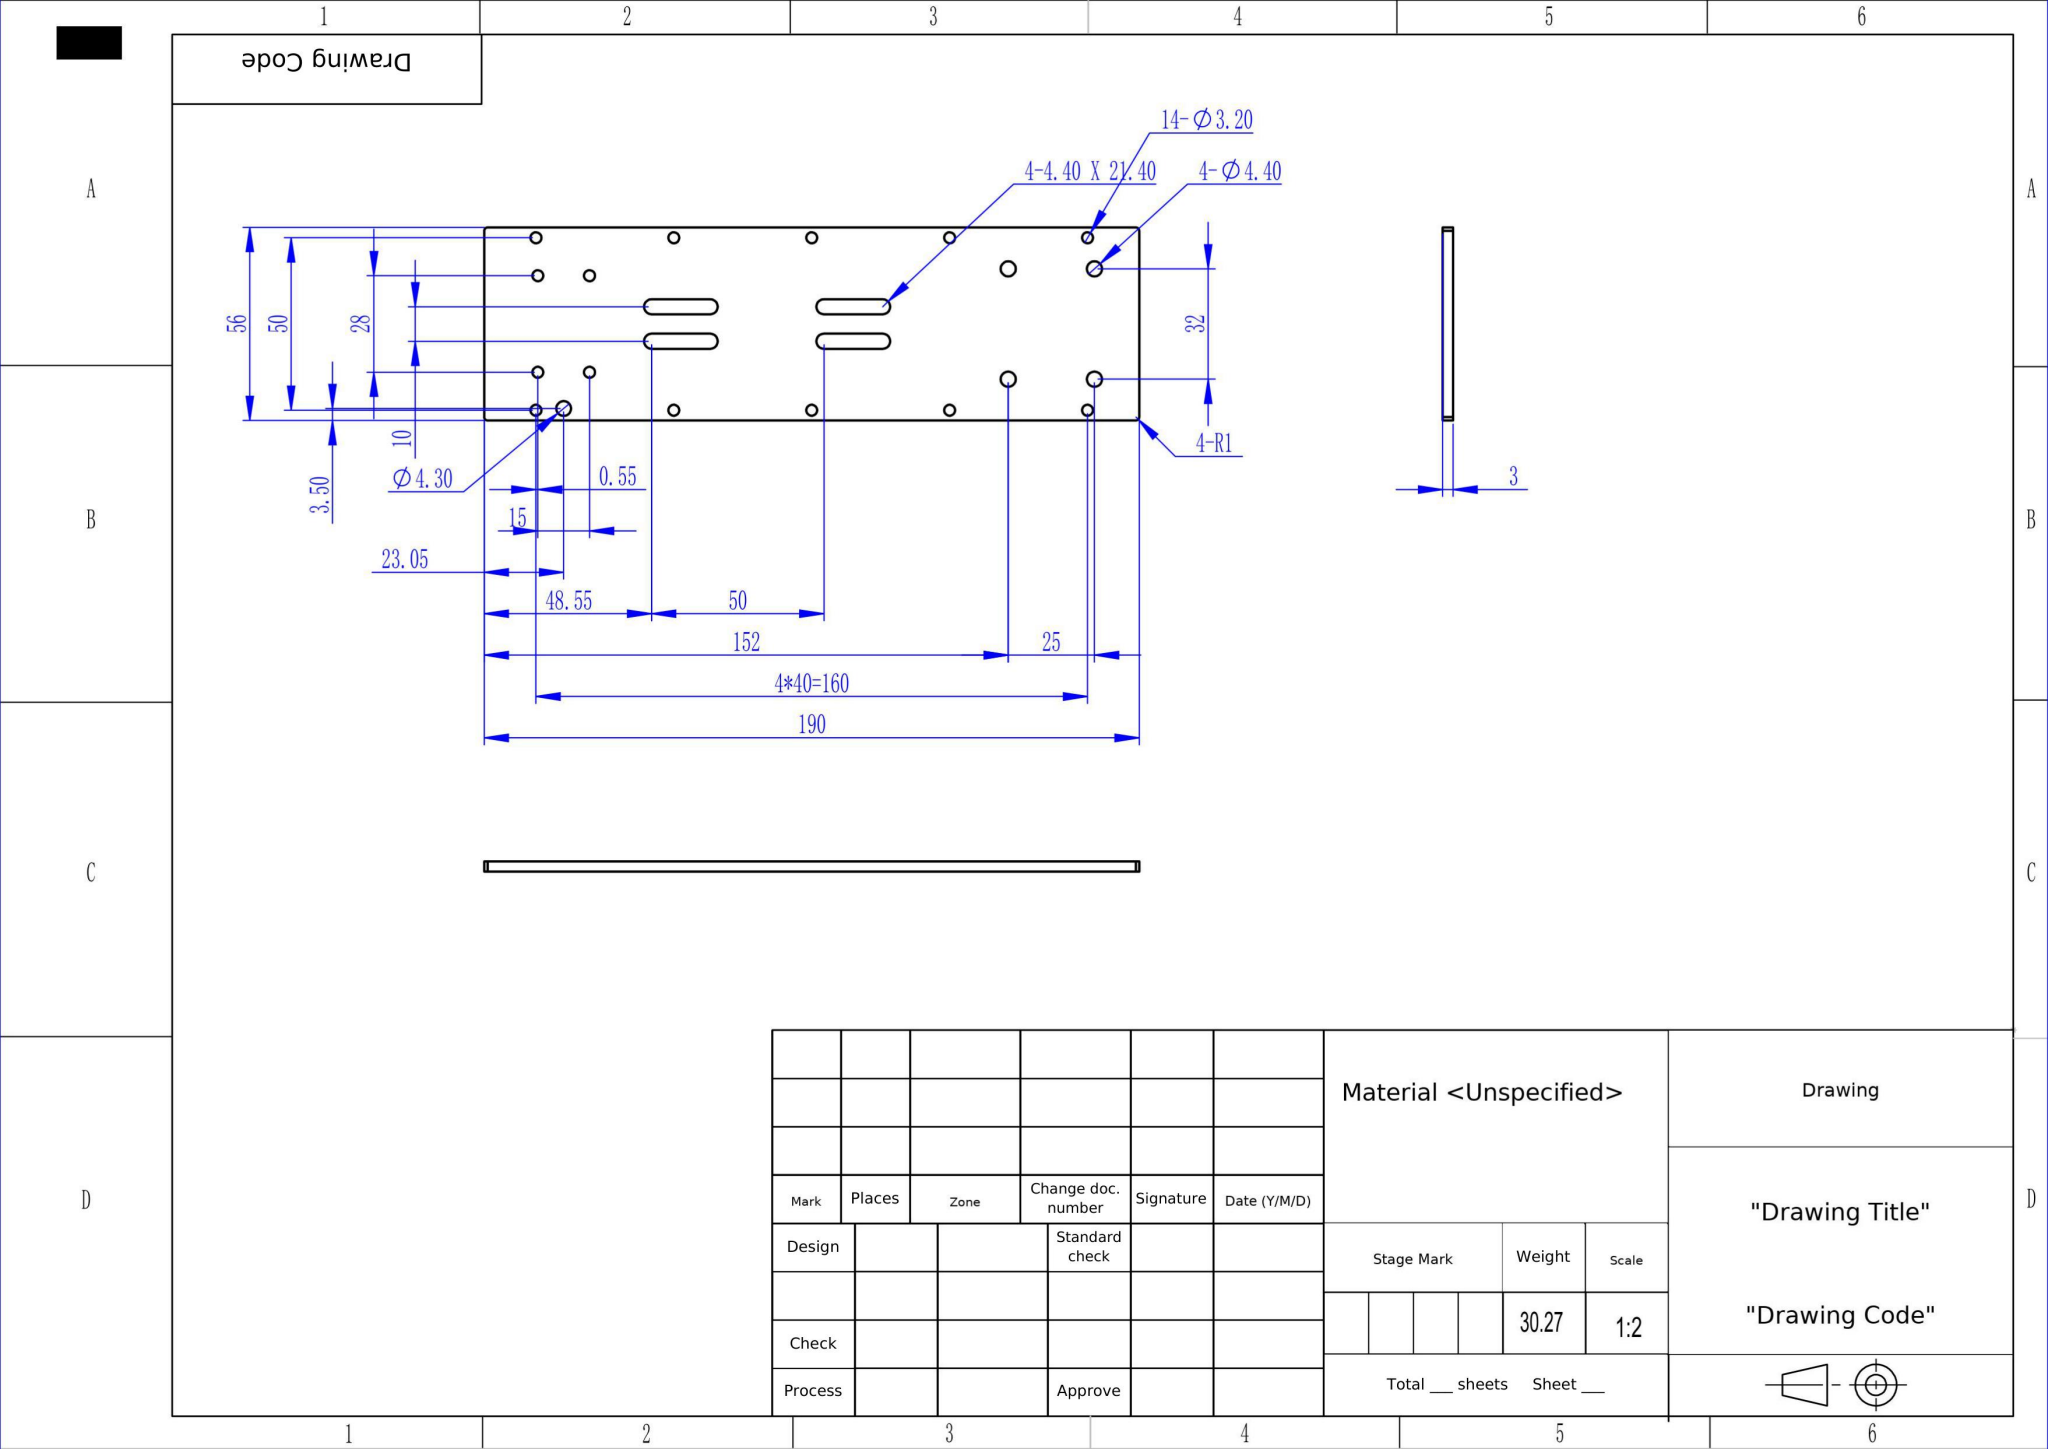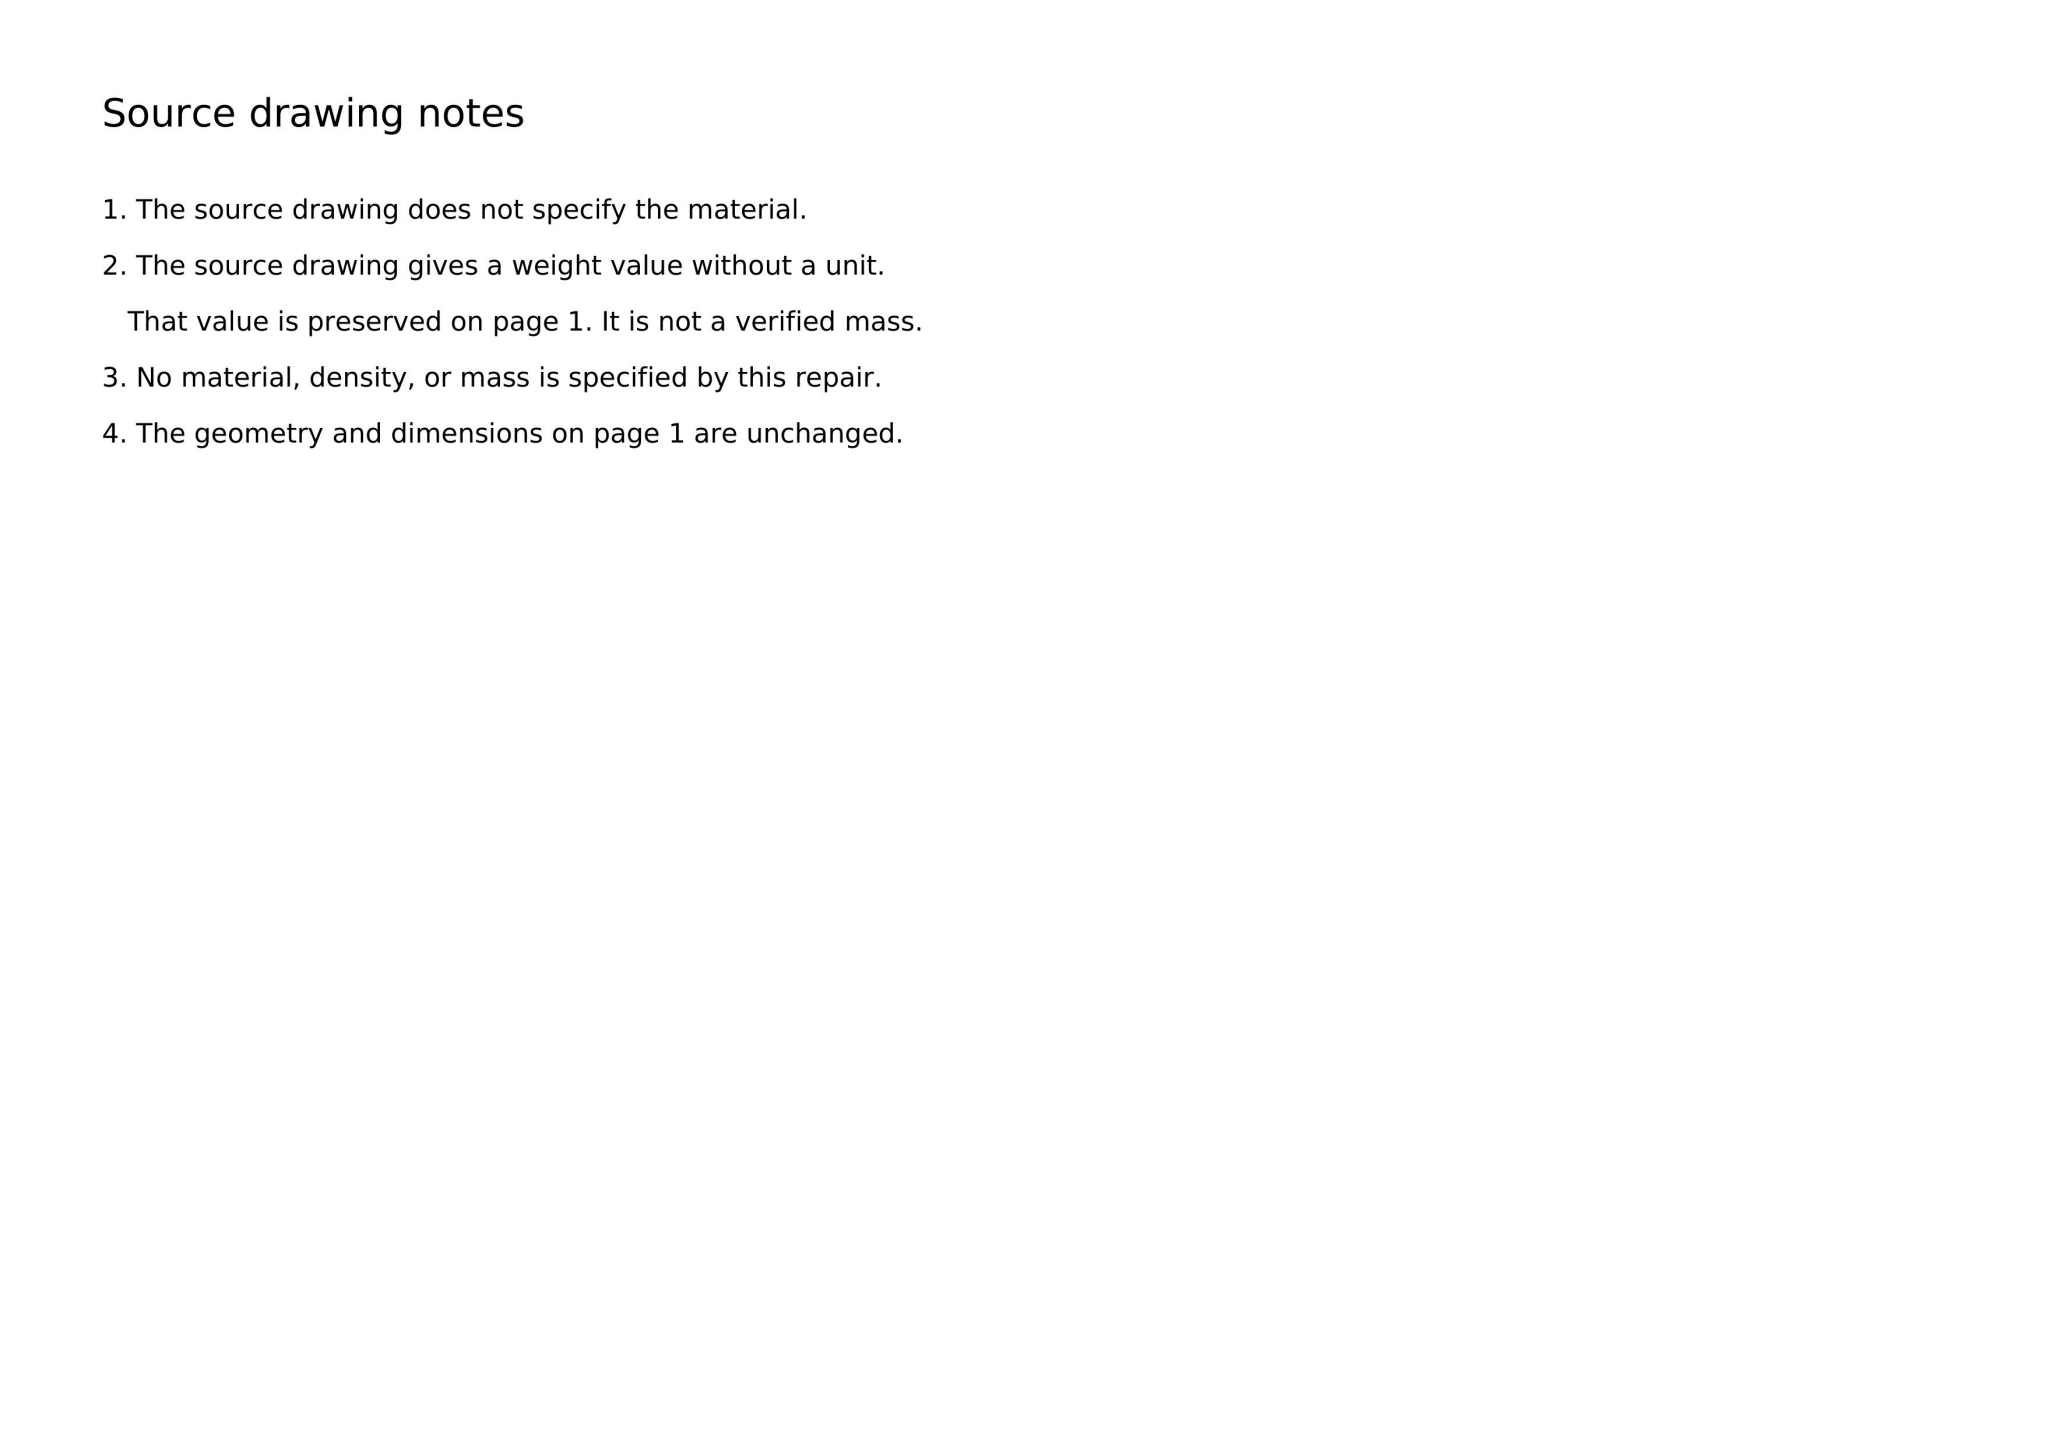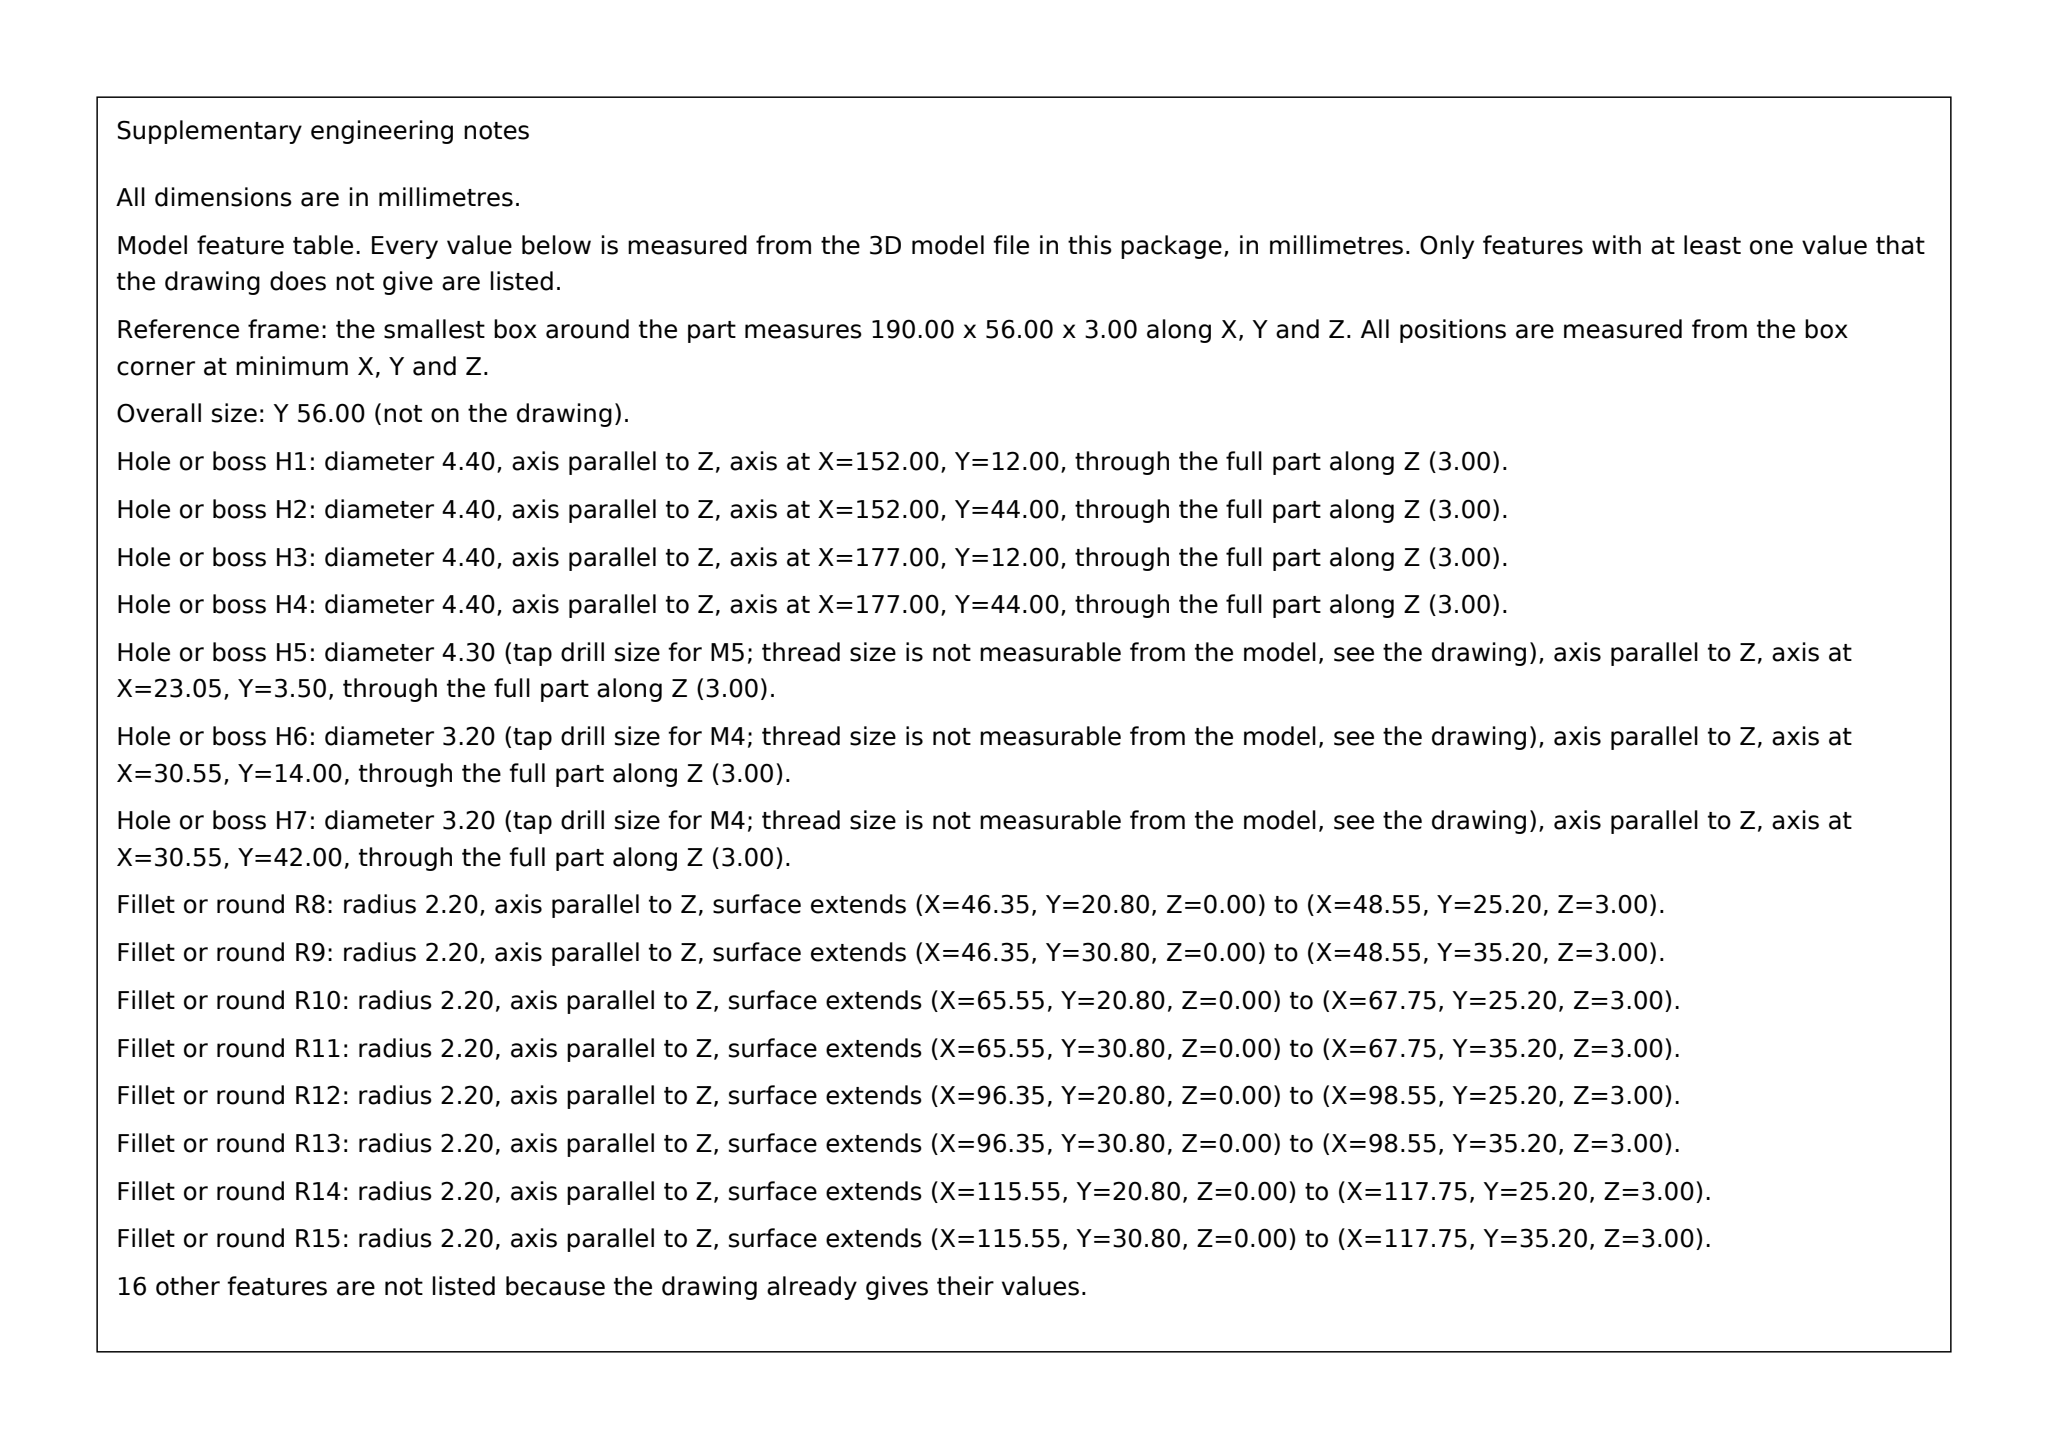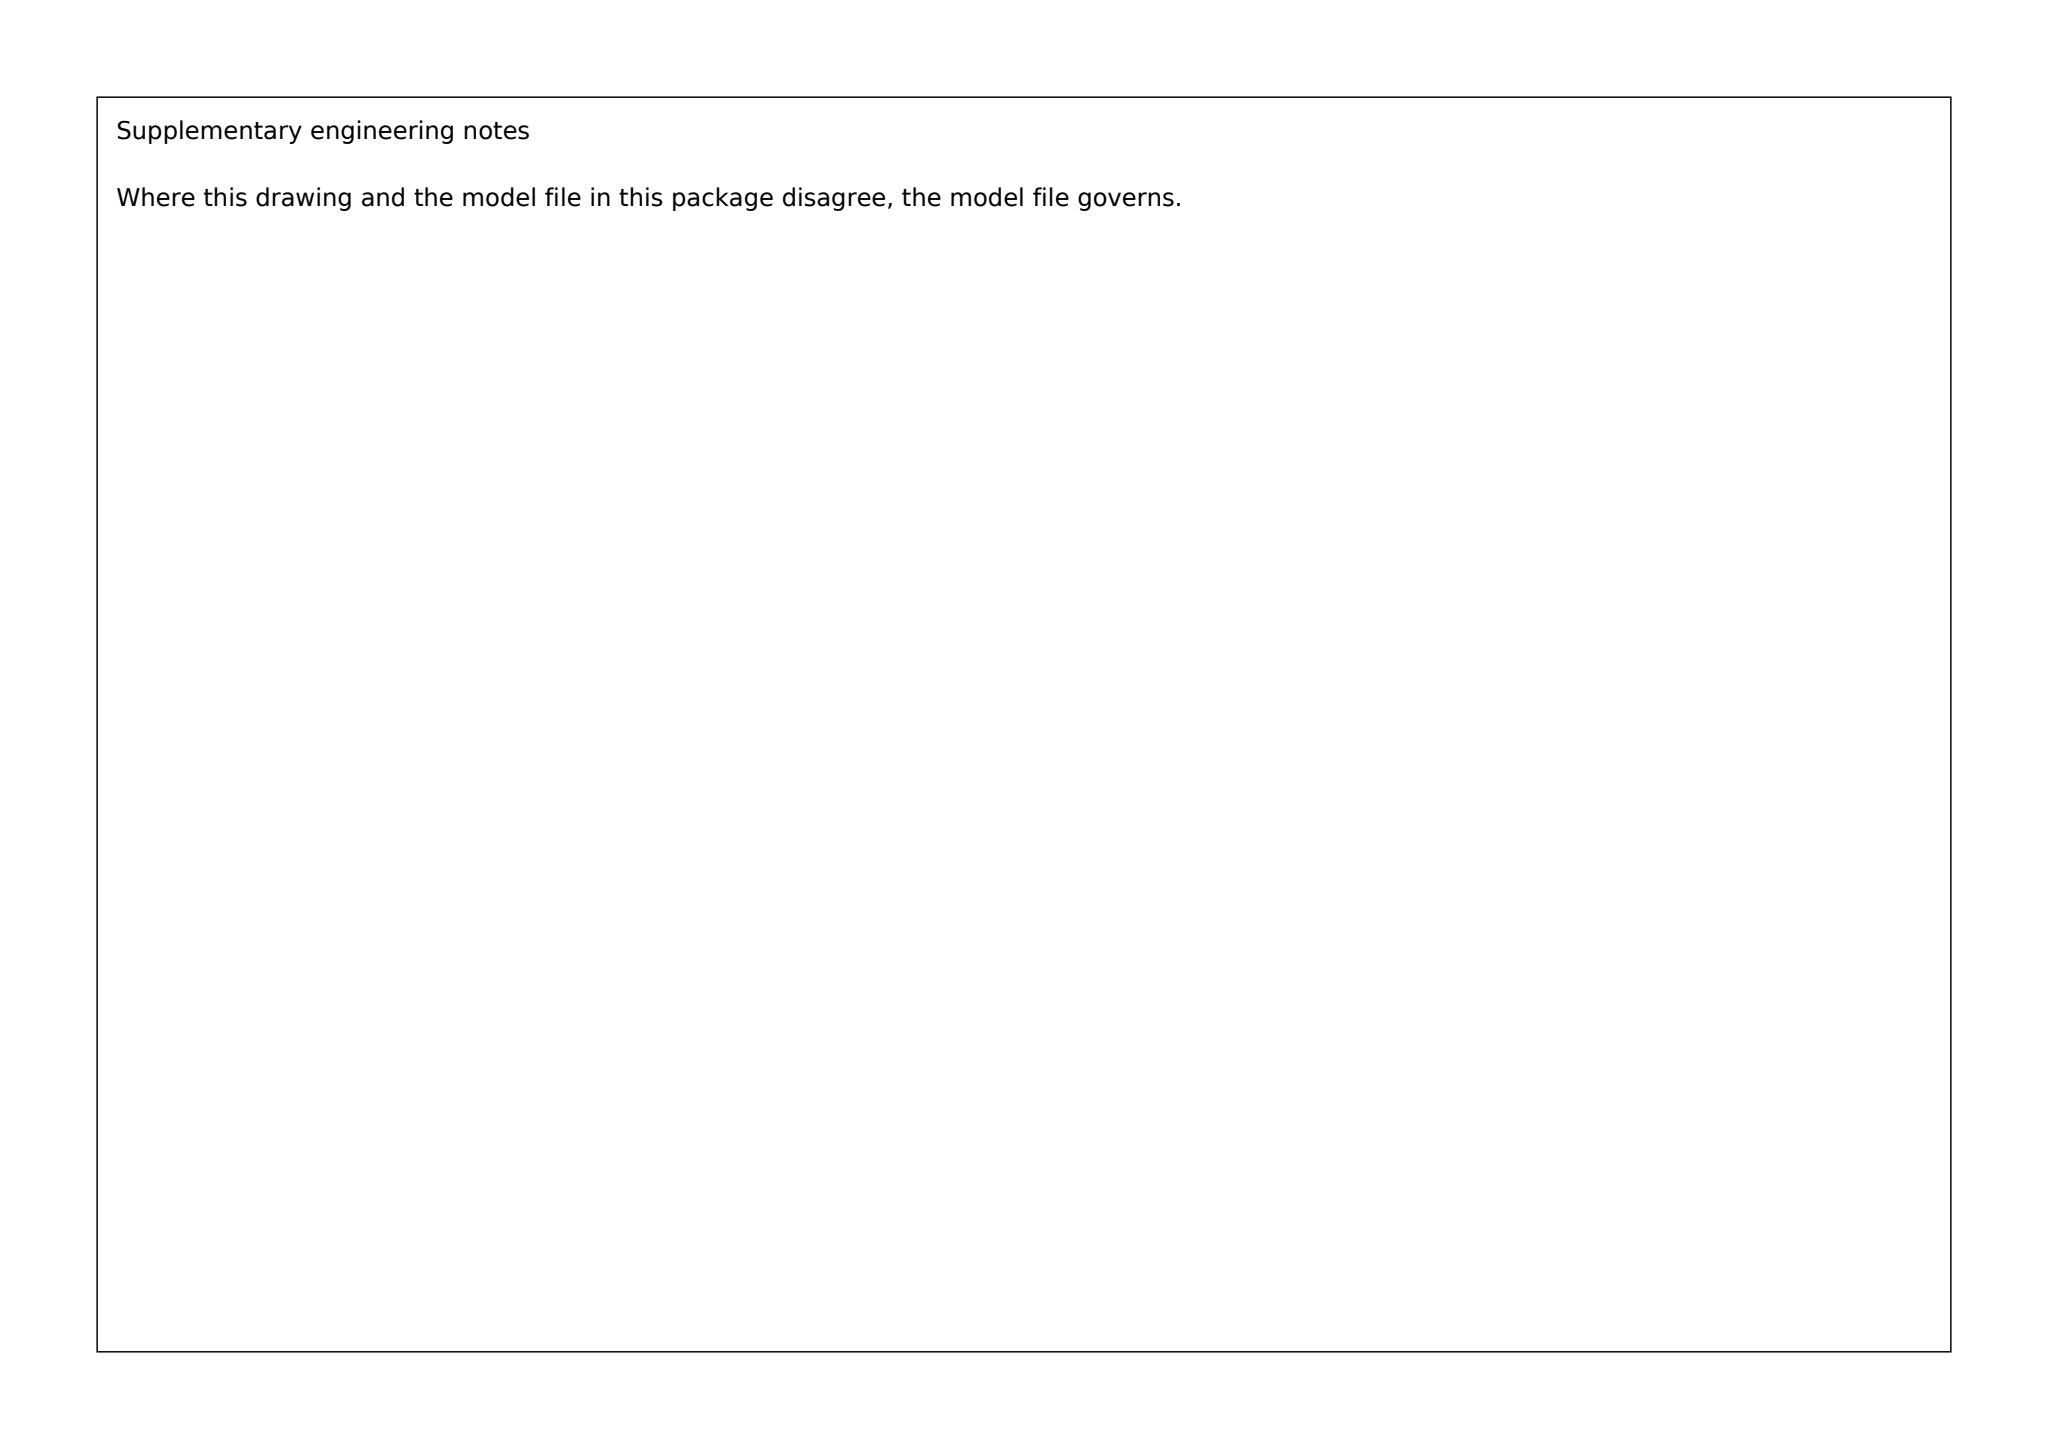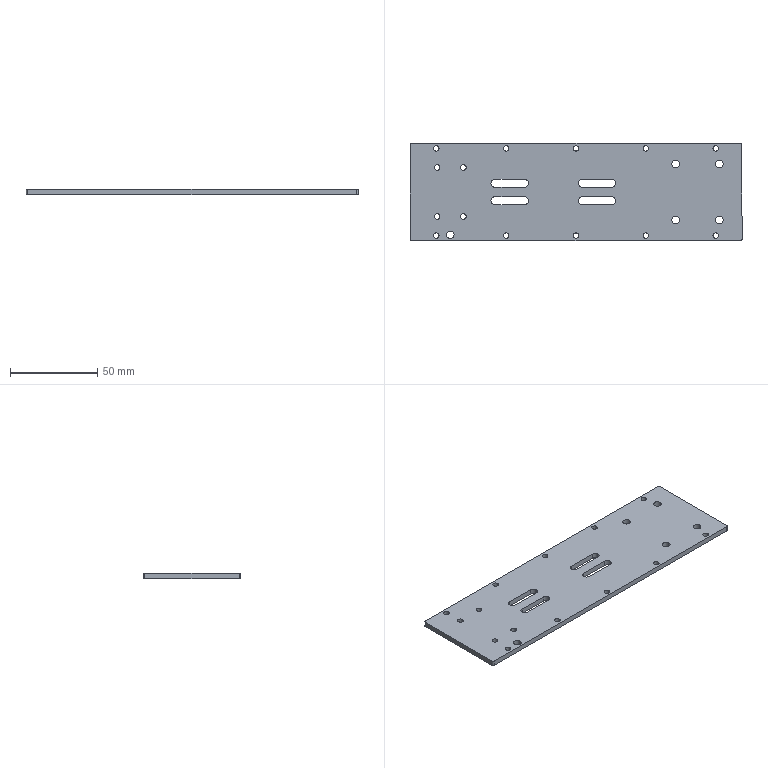Part | SolidWorks | mm | 1 solid | 72 faces | box 190 x 56 x 3 mm | volume 30274 mm3 | cylinder 58 | plane 14 | commonest cylinder face diameters 3.2 x28 4.4 x24 2 x4 4.3 x2
build123d program:
from build123d import *

# Parameters (mm, degrees)
SKETCH1_W           = 190
SKETCH1_H           = 56
SKETCH1_R           = 1.6
SKETCH1_R_2         = 2.2
SKETCH1_R_3         = 2.15
BOSS_EXTRUDE1_DEPTH = 3
FILLET1_R           = 1
CUT_EXTRUDE1_DEPTH  = 193.076


with BuildPart() as part:
    # Sketch1 → Boss-Extrude1 (new body)
    with BuildSketch(Plane.XY):
        with Locations((95, 0)):
            Rectangle(SKETCH1_W, SKETCH1_H)
        with Locations((30.55, 14)):
            Circle(SKETCH1_R, mode=Mode.SUBTRACT)
        with Locations((15.55, 14)):
            Circle(SKETCH1_R, mode=Mode.SUBTRACT)
        with Locations((15.55, -14)):
            Circle(SKETCH1_R, mode=Mode.SUBTRACT)
        with Locations((30.55, -14)):
            Circle(SKETCH1_R, mode=Mode.SUBTRACT)
        with Locations((177, 16)):
            Circle(SKETCH1_R_2, mode=Mode.SUBTRACT)
        with Locations((152, 16)):
            Circle(SKETCH1_R_2, mode=Mode.SUBTRACT)
        with Locations((152, -16)):
            Circle(SKETCH1_R_2, mode=Mode.SUBTRACT)
        with Locations((177, -16)):
            Circle(SKETCH1_R_2, mode=Mode.SUBTRACT)
        with Locations((48.55, 5)):
            Circle(SKETCH1_R_2, mode=Mode.SUBTRACT)
        with Locations((48.55, -5)):
            Circle(SKETCH1_R_2, mode=Mode.SUBTRACT)
        with Locations((98.55, -5)):
            Circle(SKETCH1_R_2, mode=Mode.SUBTRACT)
        with Locations((98.55, 5)):
            Circle(SKETCH1_R_2, mode=Mode.SUBTRACT)
        with Locations((15, 25)):
            Circle(SKETCH1_R, mode=Mode.SUBTRACT)
        with Locations((55, 25)):
            Circle(SKETCH1_R, mode=Mode.SUBTRACT)
        with Locations((95, 25)):
            Circle(SKETCH1_R, mode=Mode.SUBTRACT)
        with Locations((135, 25)):
            Circle(SKETCH1_R, mode=Mode.SUBTRACT)
        with Locations((175, 25)):
            Circle(SKETCH1_R, mode=Mode.SUBTRACT)
        with Locations((15, -25)):
            Circle(SKETCH1_R, mode=Mode.SUBTRACT)
        with Locations((55, -25)):
            Circle(SKETCH1_R, mode=Mode.SUBTRACT)
        with Locations((95, -25)):
            Circle(SKETCH1_R, mode=Mode.SUBTRACT)
        with Locations((135, -25)):
            Circle(SKETCH1_R, mode=Mode.SUBTRACT)
        with Locations((175, -25)):
            Circle(SKETCH1_R, mode=Mode.SUBTRACT)
        with Locations((23.05, -24.5)):
            Circle(SKETCH1_R_3, mode=Mode.SUBTRACT)
    extrude(amount=BOSS_EXTRUDE1_DEPTH)

    # Fillet1
    fillet1_edges = [part.edges().sort_by_distance(p)[0] for p in [
        (0, 28, 1.5),
        (190, 28, 1.5),
        (190, -28, 1.5),
        (0, -28, 1.5),
    ]]
    fillet(fillet1_edges, radius=FILLET1_R)

    # Sketch2 → Cut-Extrude1 (cut, through all)
    with BuildSketch(Plane.XY.offset(3)):
        with BuildLine():
            Line((48.55, 7.2), (65.55, 7.2))
            ThreePointArc((65.55, 7.2), (67.75, 5), (65.55, 2.8))
            Line((65.55, 2.8), (48.55, 2.8))
            ThreePointArc((48.55, 2.8), (46.35, 5), (48.55, 7.2))
        make_face()
        with BuildLine():
            Line((48.55, -2.8), (65.55, -2.8))
            ThreePointArc((65.55, -2.8), (67.75, -5), (65.55, -7.2))
            Line((65.55, -7.2), (48.55, -7.2))
            ThreePointArc((48.55, -7.2), (46.35, -5), (48.55, -2.8))
        make_face()
        with BuildLine():
            Line((98.55, 7.2), (115.55, 7.2))
            ThreePointArc((115.55, 7.2), (117.75, 5), (115.55, 2.8))
            Line((115.55, 2.8), (98.55, 2.8))
            ThreePointArc((98.55, 2.8), (96.35, 5), (98.55, 7.2))
        make_face()
        with BuildLine():
            Line((98.55, -2.8), (115.55, -2.8))
            ThreePointArc((115.55, -2.8), (117.75, -5), (115.55, -7.2))
            Line((115.55, -7.2), (98.55, -7.2))
            ThreePointArc((98.55, -7.2), (96.35, -5), (98.55, -2.8))
        make_face()
    extrude(amount=-CUT_EXTRUDE1_DEPTH, mode=Mode.SUBTRACT)


solid = part.part